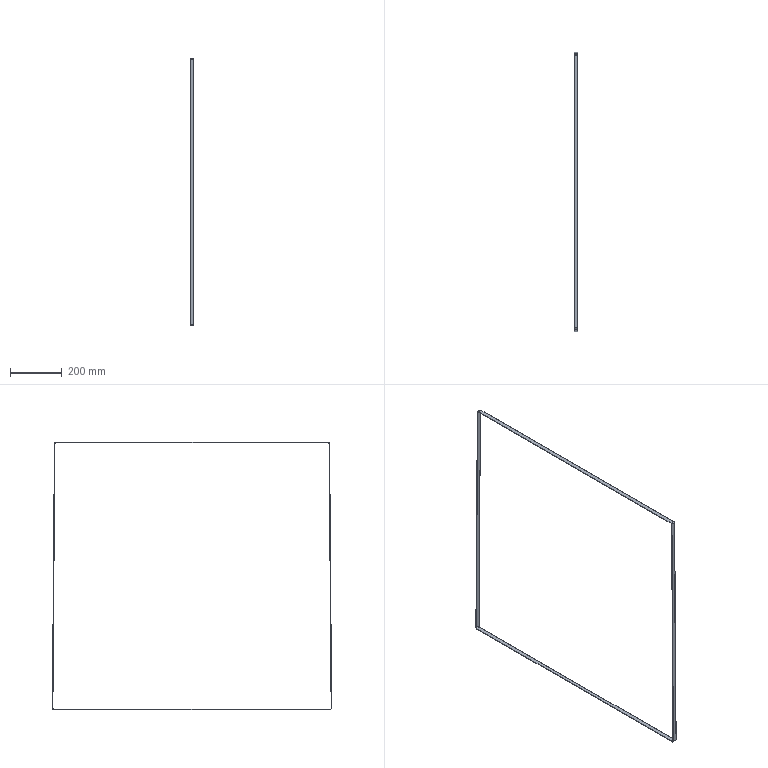Component | NX | SHORT_PACKAGING_STRAP | 1 solid | 18 faces | volume 125227 mm3 | plane 12 | cylinder 6 | commonest cylinder face diameters 10 x3 6 x3